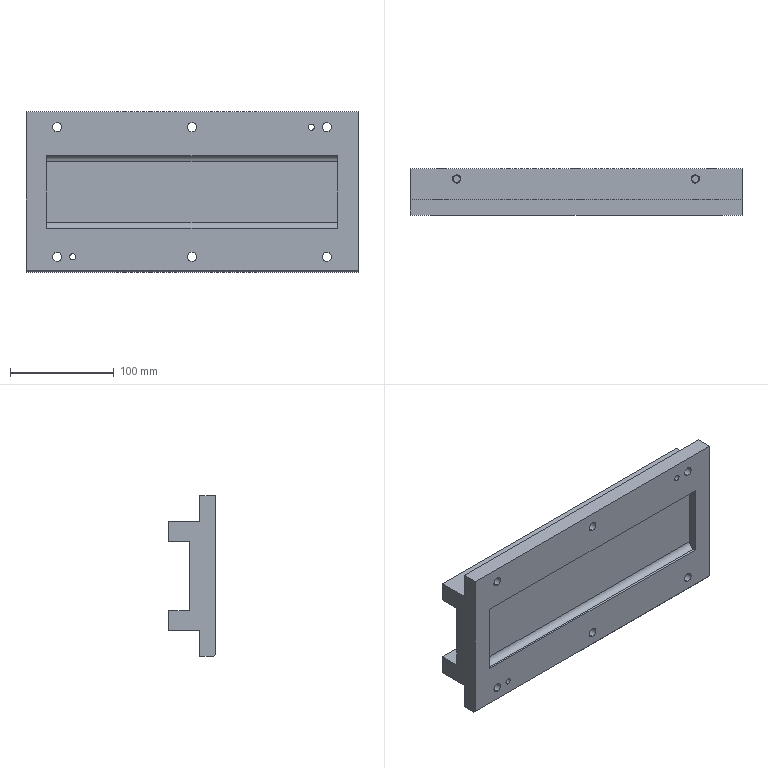Component | SolidWorks | 24FixtureBase-1 | 1 solid | 100 faces | volume 1152602 mm3 | cylinder 46 | cone 28 | plane 26 | commonest cylinder face diameters 6.8 x16 14 x12 9 x12 6 x4 12 x2